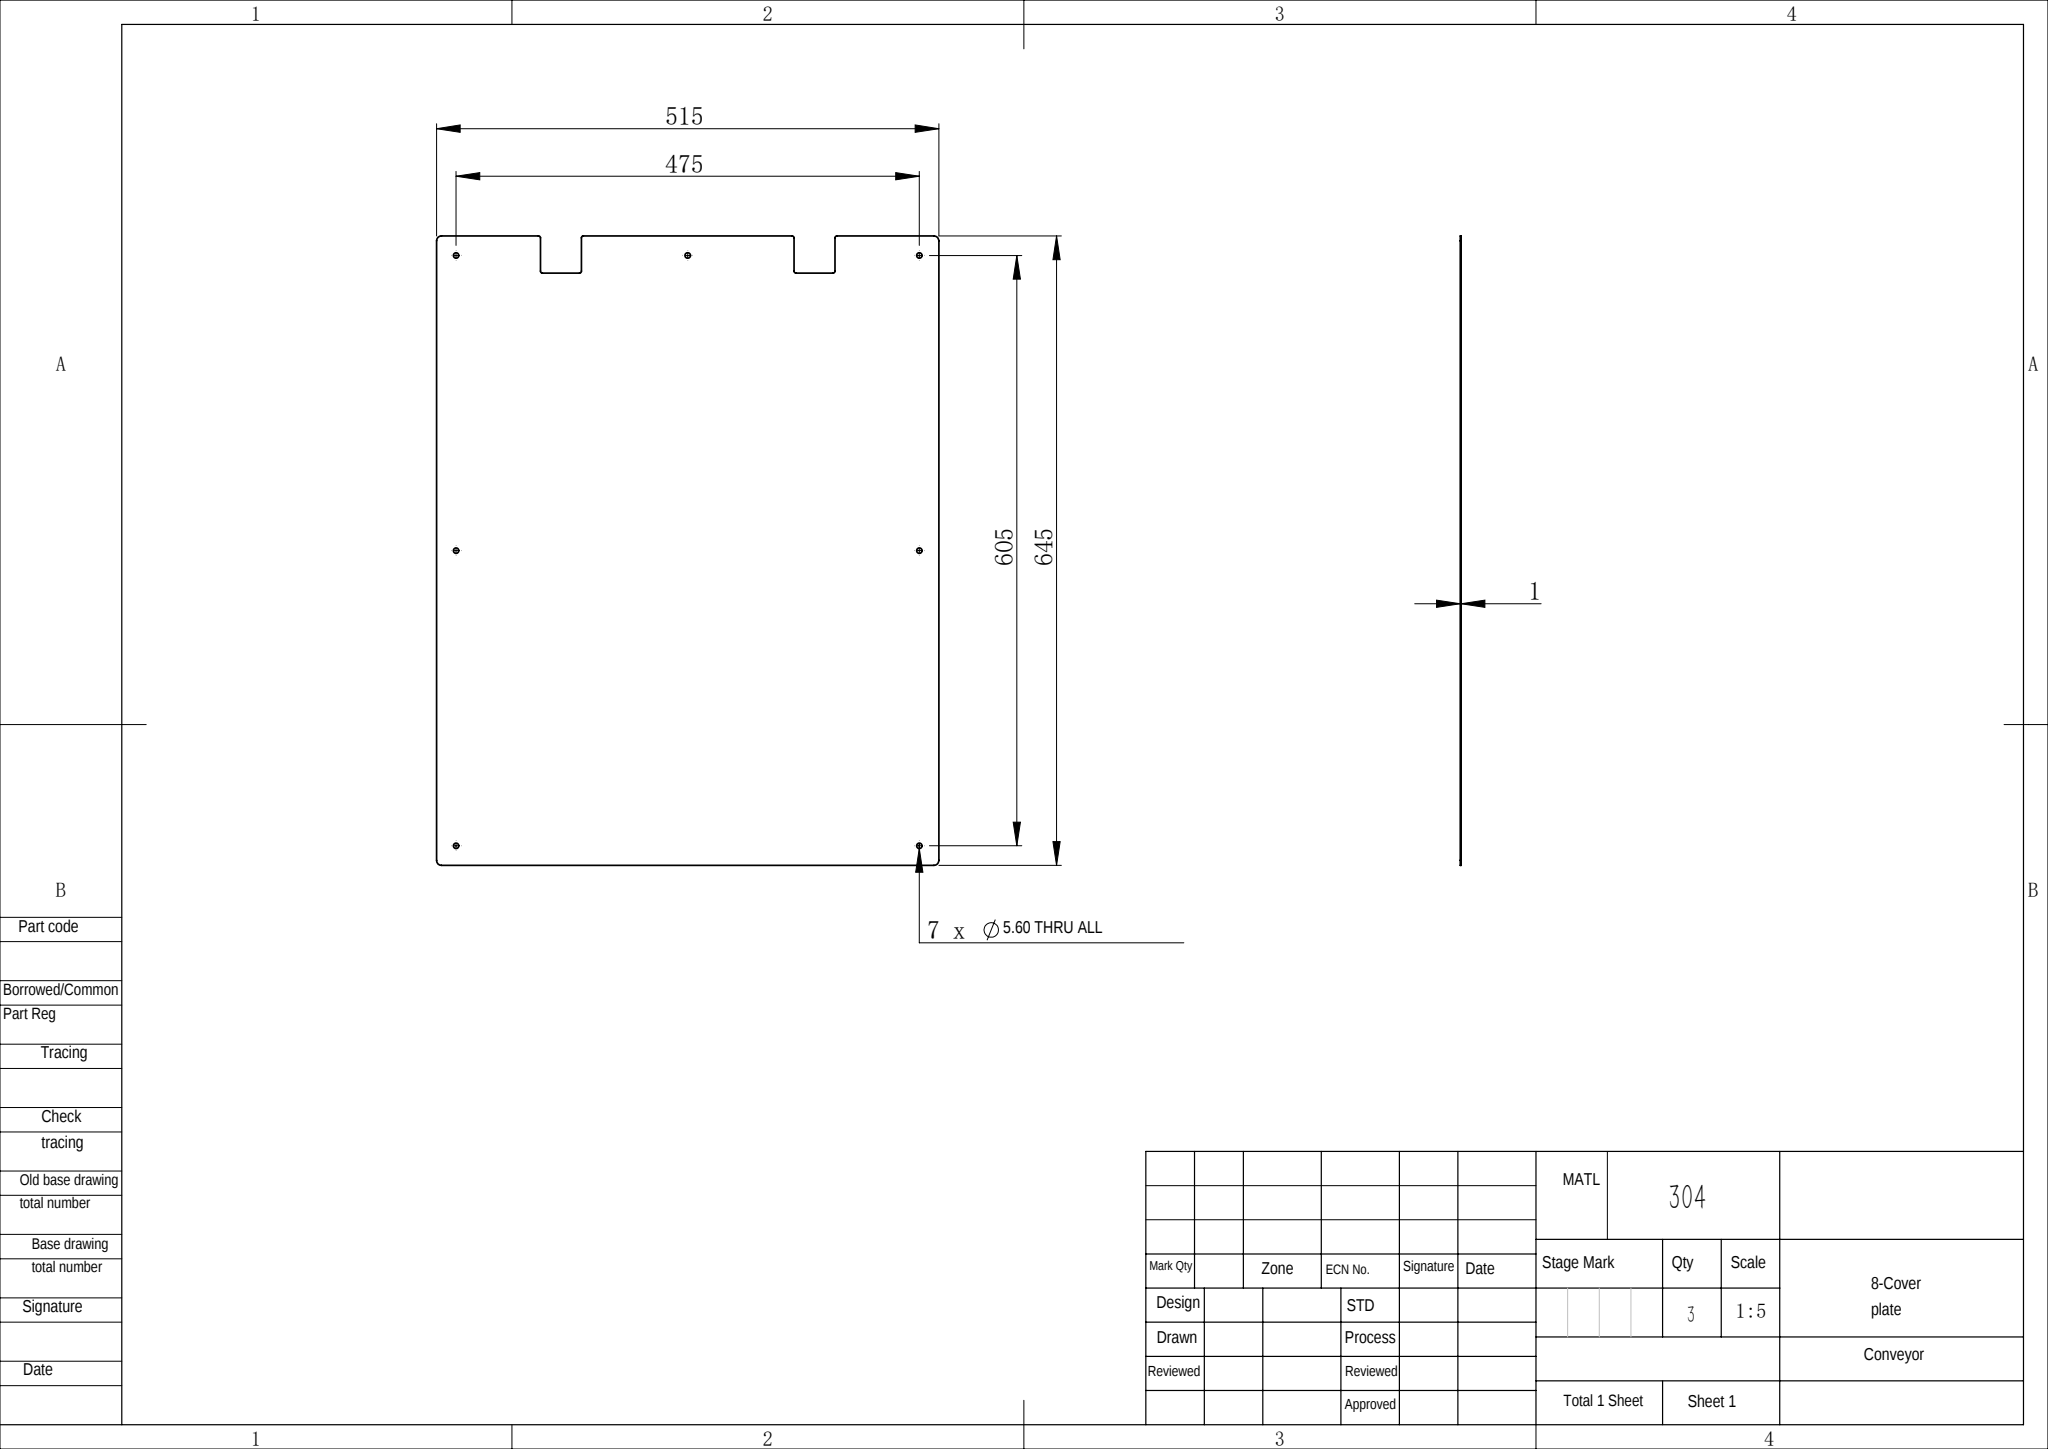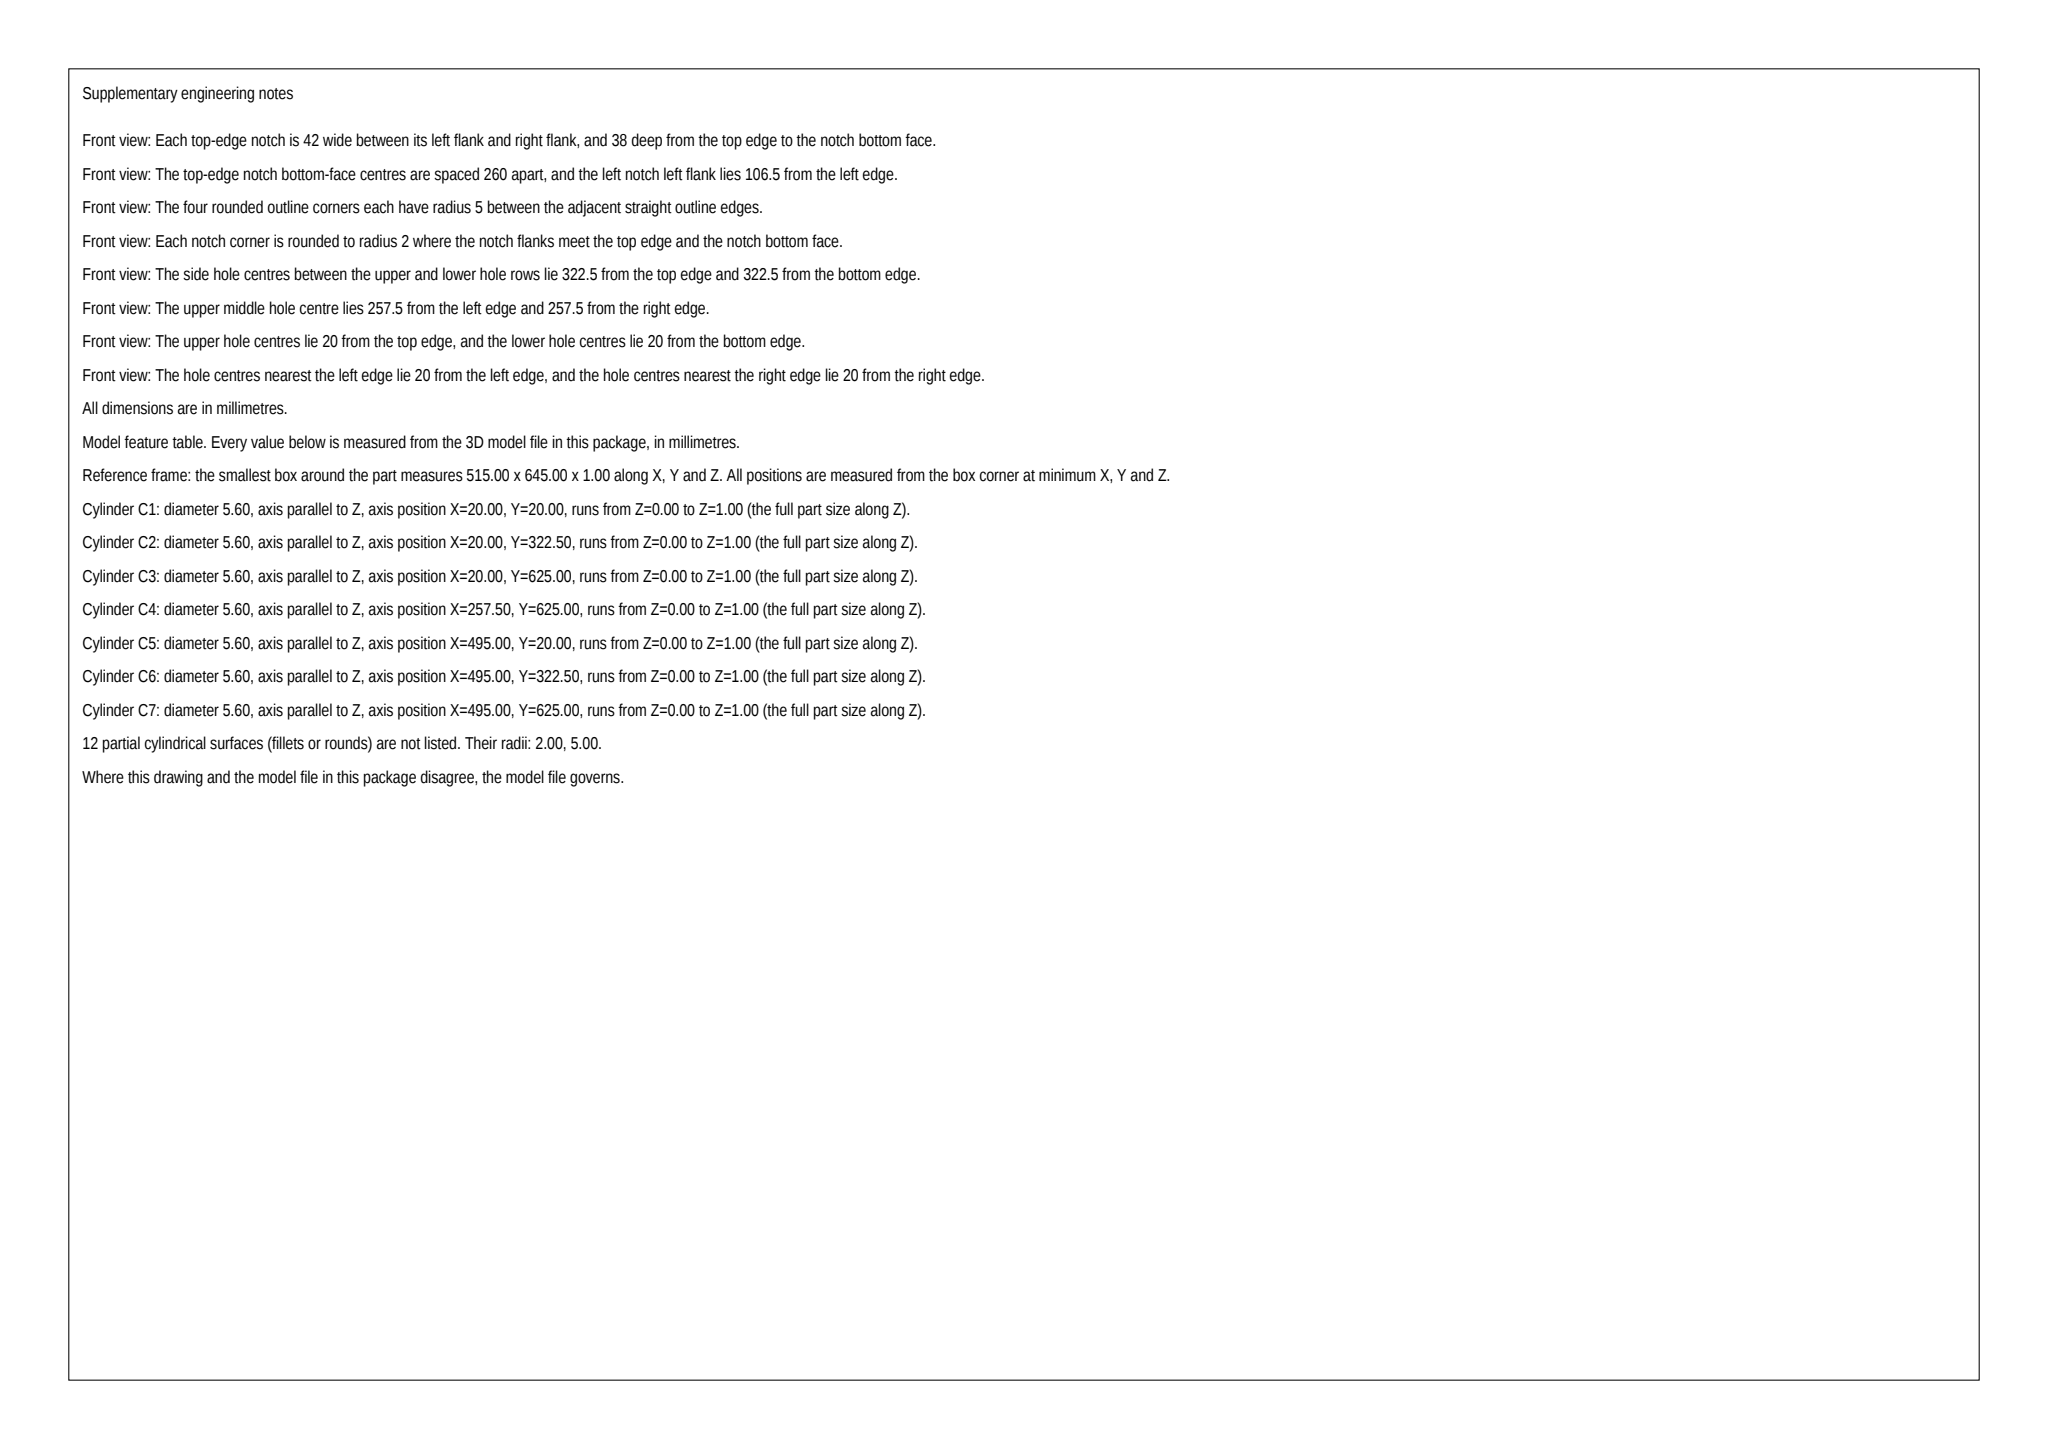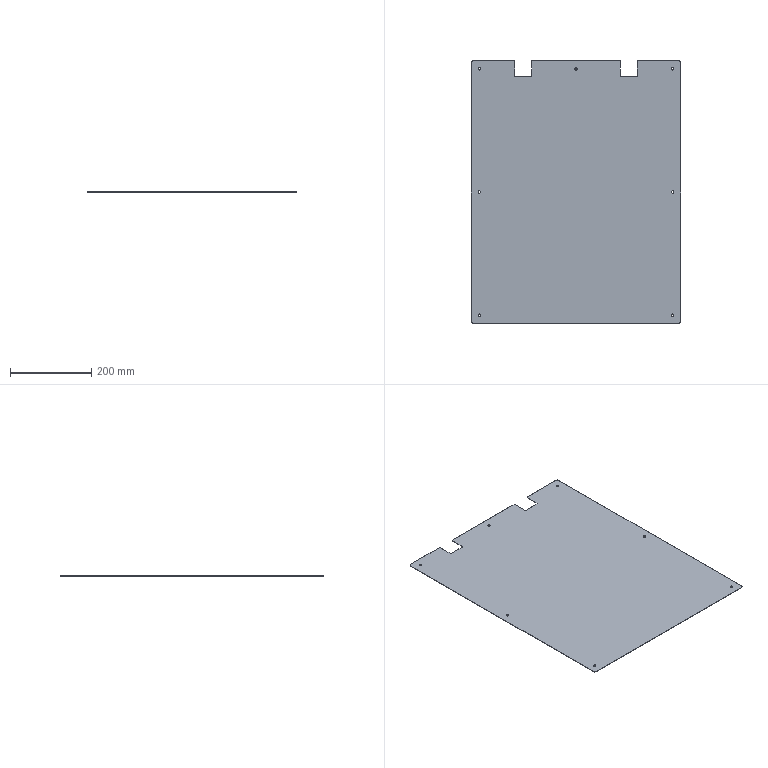Part | SolidWorks | mm | 1 solid | 40 faces | box 515 x 645 x 1 mm | volume 328789 mm3 | cylinder 26 | plane 14 | commonest cylinder face diameters 5.6 x14 4 x8 10 x4
Drawing notes:
MID ROW 2X Ø5.60: 322.5 FROM BOTTOM EDGE (EQ SP, 302.5 PITCH) | from the solid: Ø5.6 holes at y=322.5 (x=20, 495); end holes y=20 & 625 (bbox Y=645)
TOP CTR Ø5.60 ON CL: 257.5 FROM LH EDGE, 625 FROM BOTTOM EDGE | from the solid: Ø5.6 hole at [257.5, 625]; bbox X=515 so x=257.5 is part CL
2X 42 NOTCHES SYM ABOUT CL: 106.5 LH EDGE TO 1ST NOTCH FACE | from the solid: notch faces x=106.5/148.5 and 366.5/408.5, 38 deep from y=645 to 607